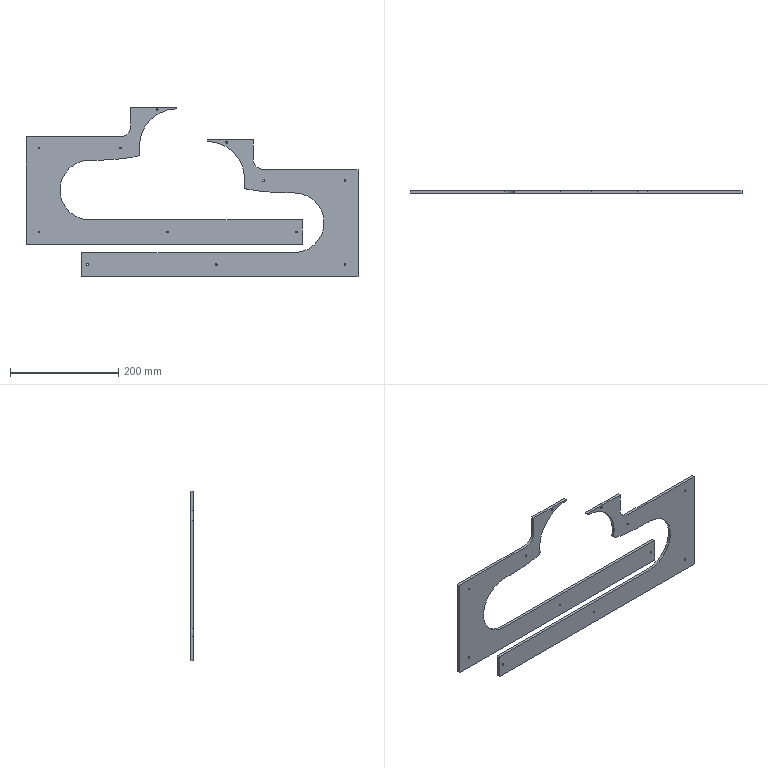CAM job | Mastercam | mm | 4 operations | part box 612.5 x 5 x 313.25
1. Contour (Ramp) | 3 - 3 平铣刀
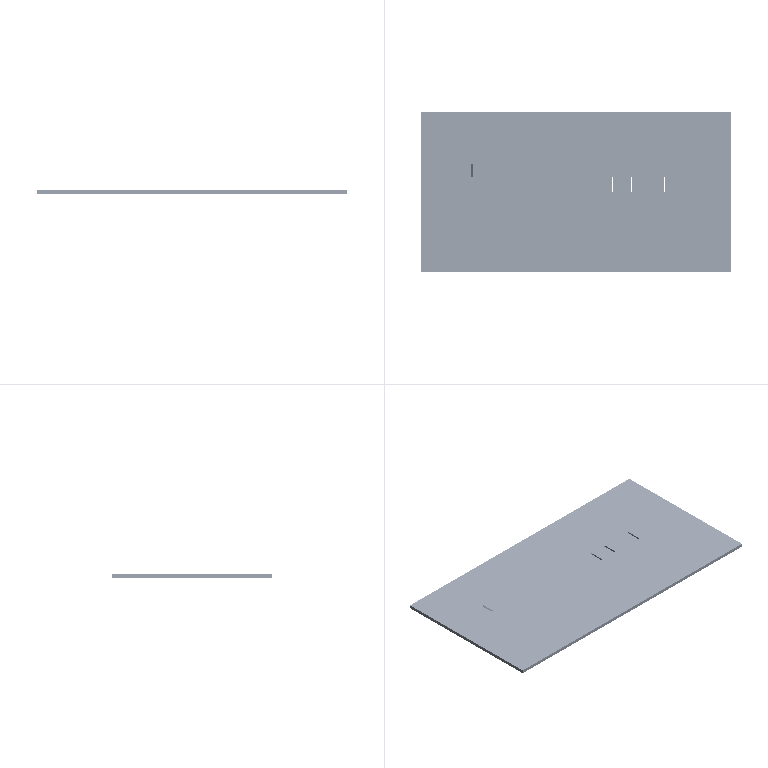2. Drill/Counterbore | 7 - 4 倒角刀
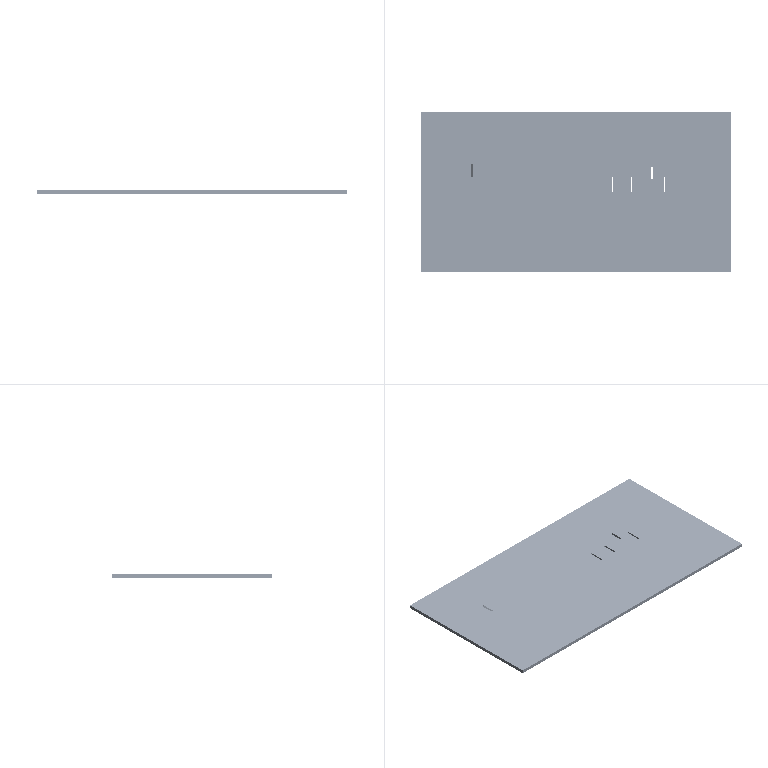3. Contour (2D chamfer) | 7 - 4 倒角刀
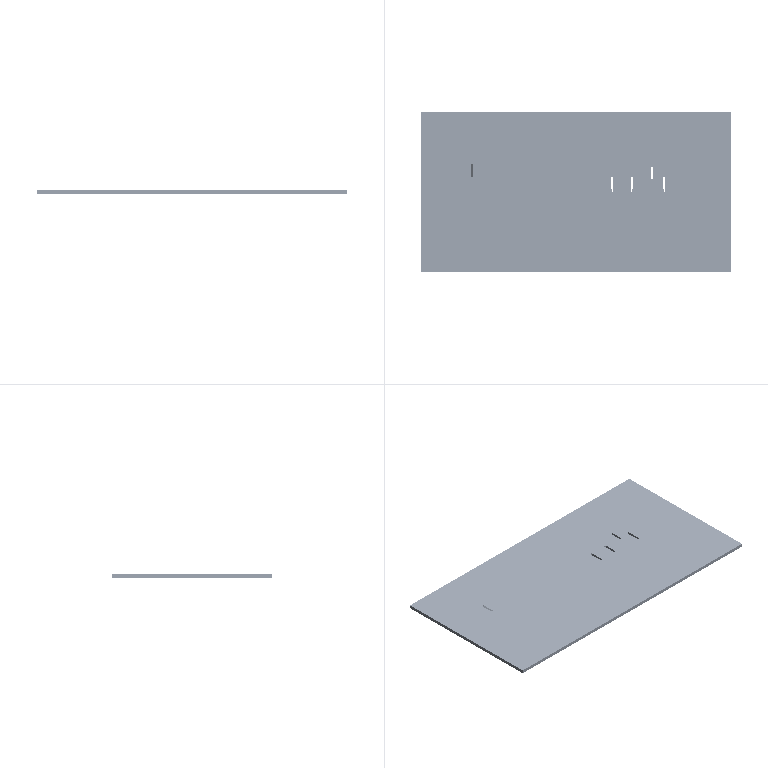4. Contour (Ramp) | 2 - 2 平铣刀